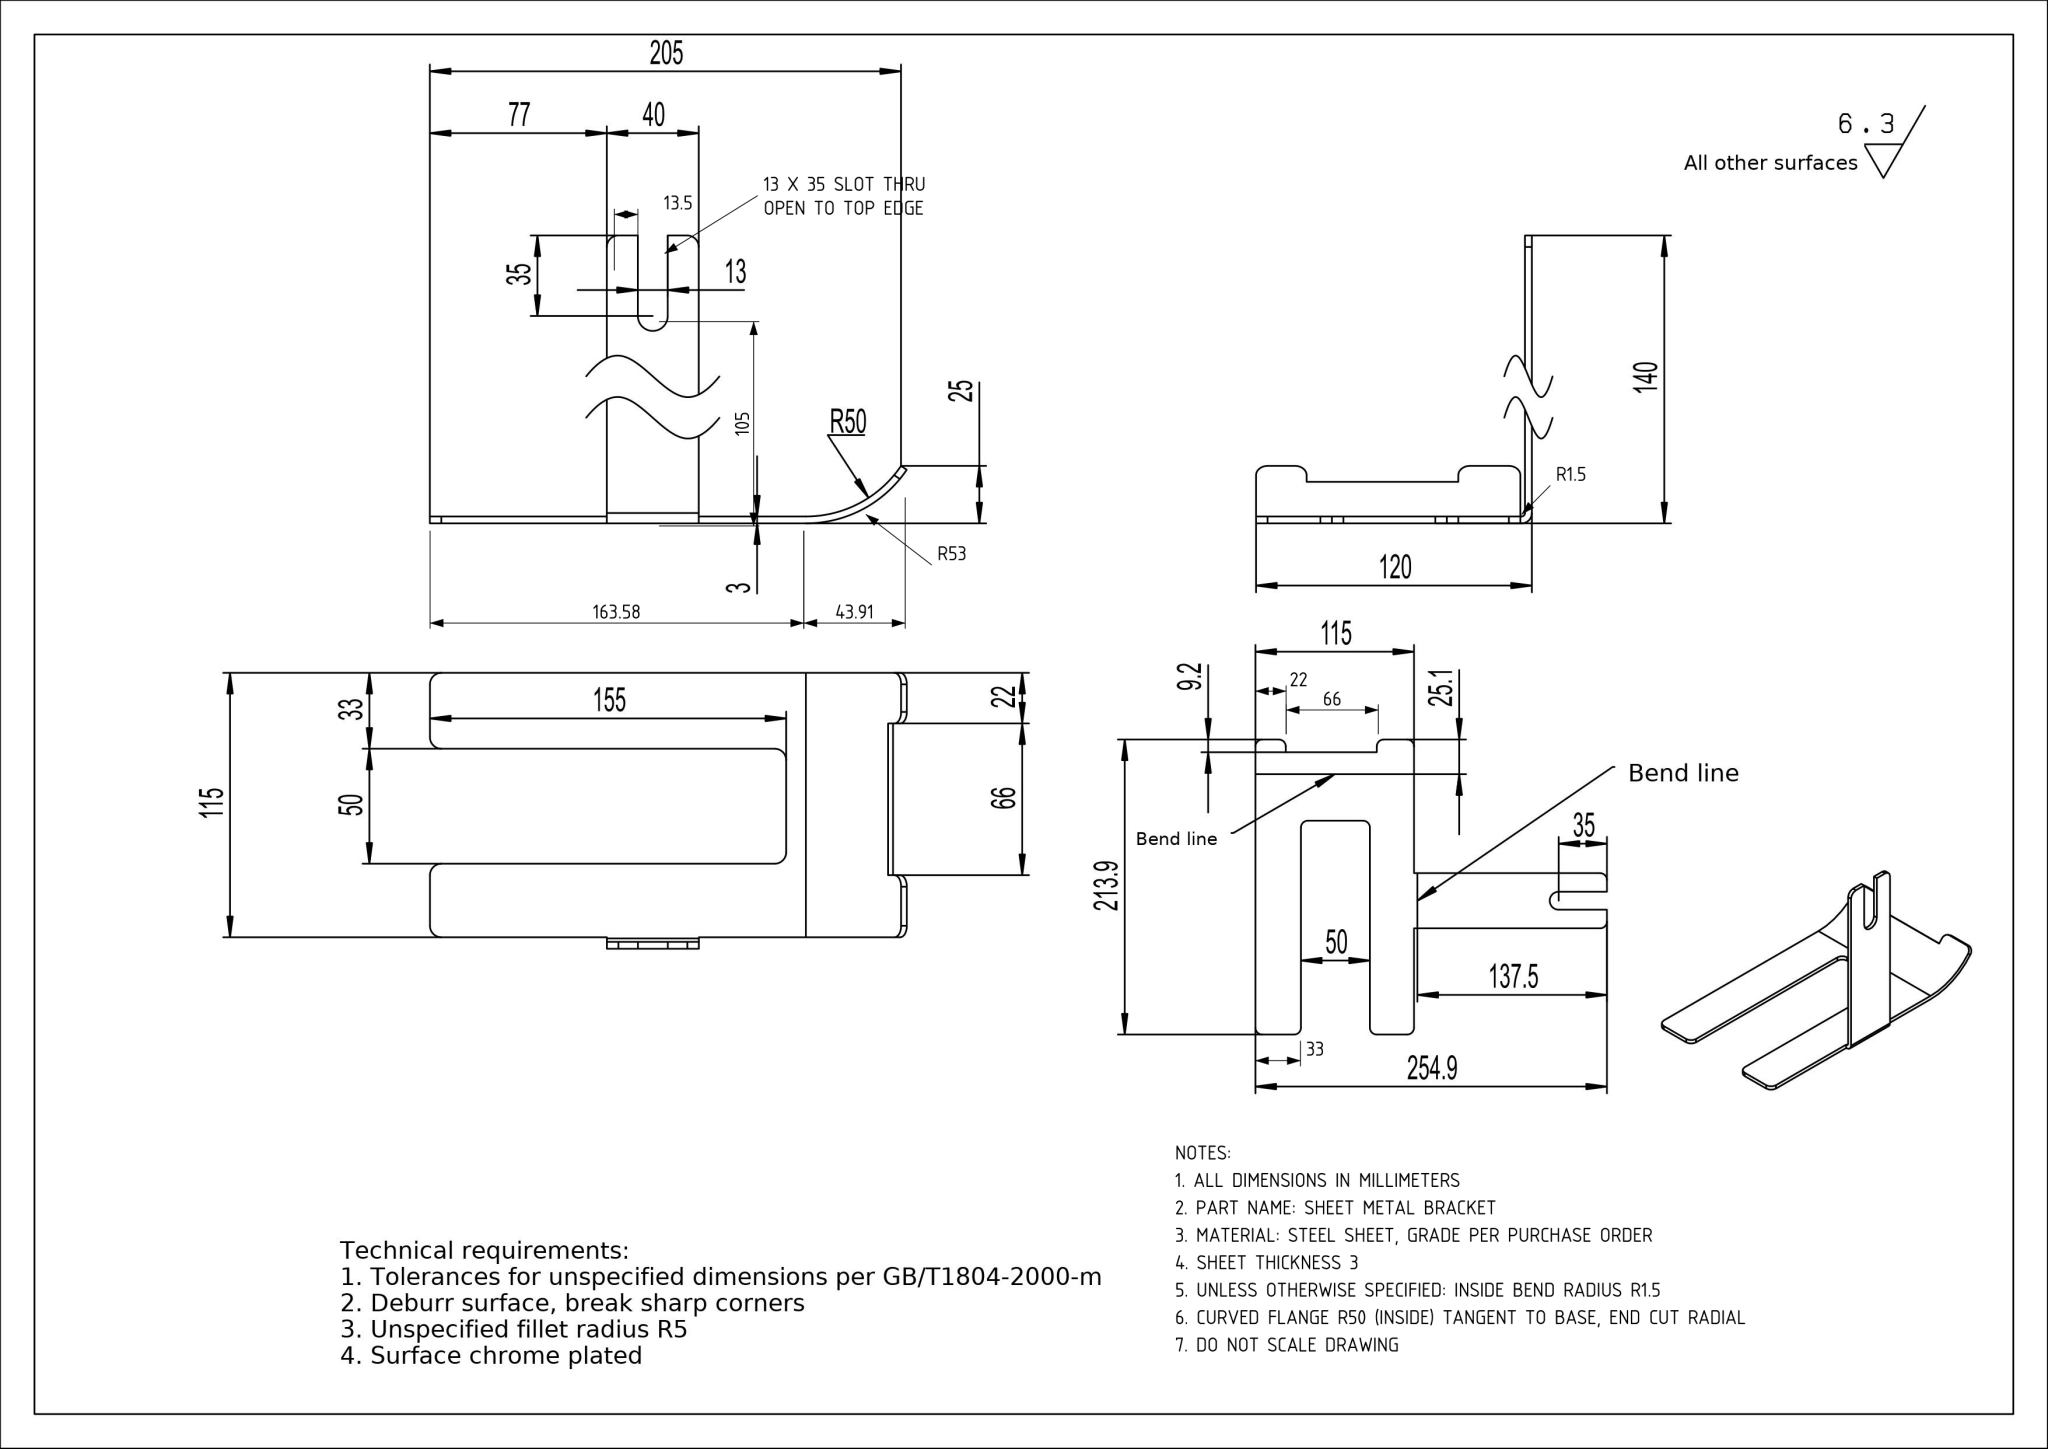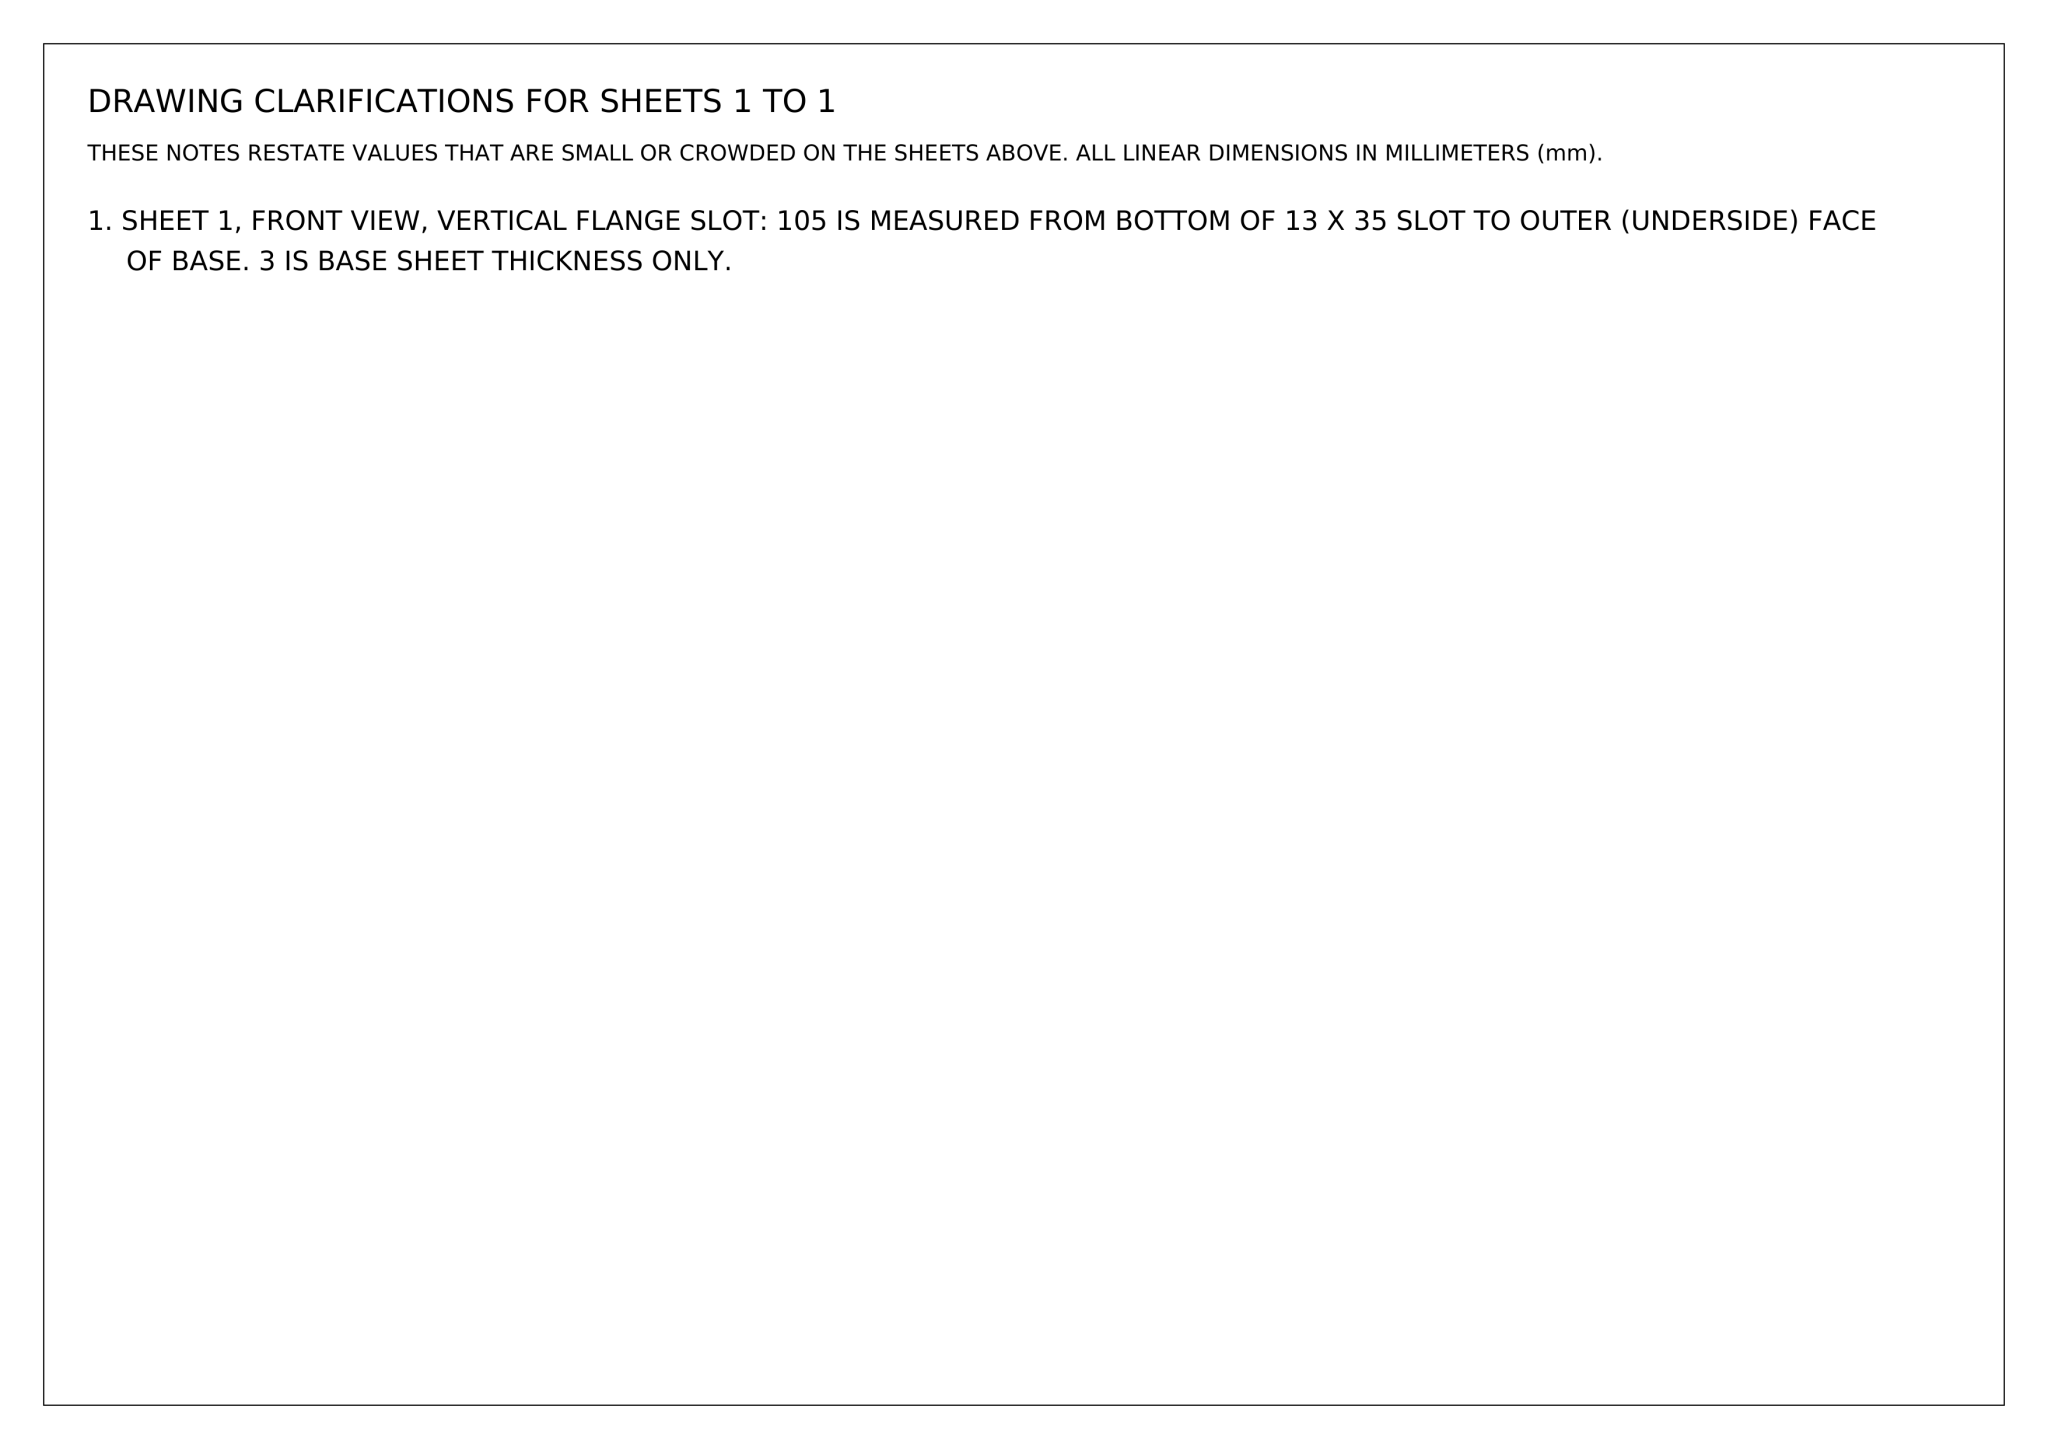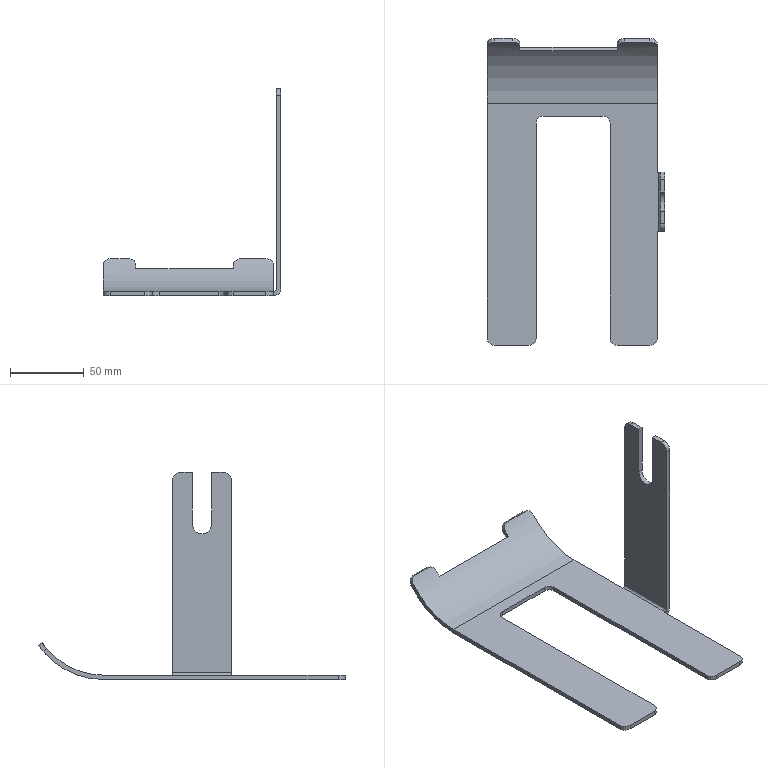Part | NX | mm | 1 solid | 40 faces | box 120 x 207.49 x 140 mm | volume 63895 mm3 | plane 23 | cylinder 17 | commonest cylinder face diameters 10 x12 100 x1 106 x1 3 x1 9 x1 13 x1